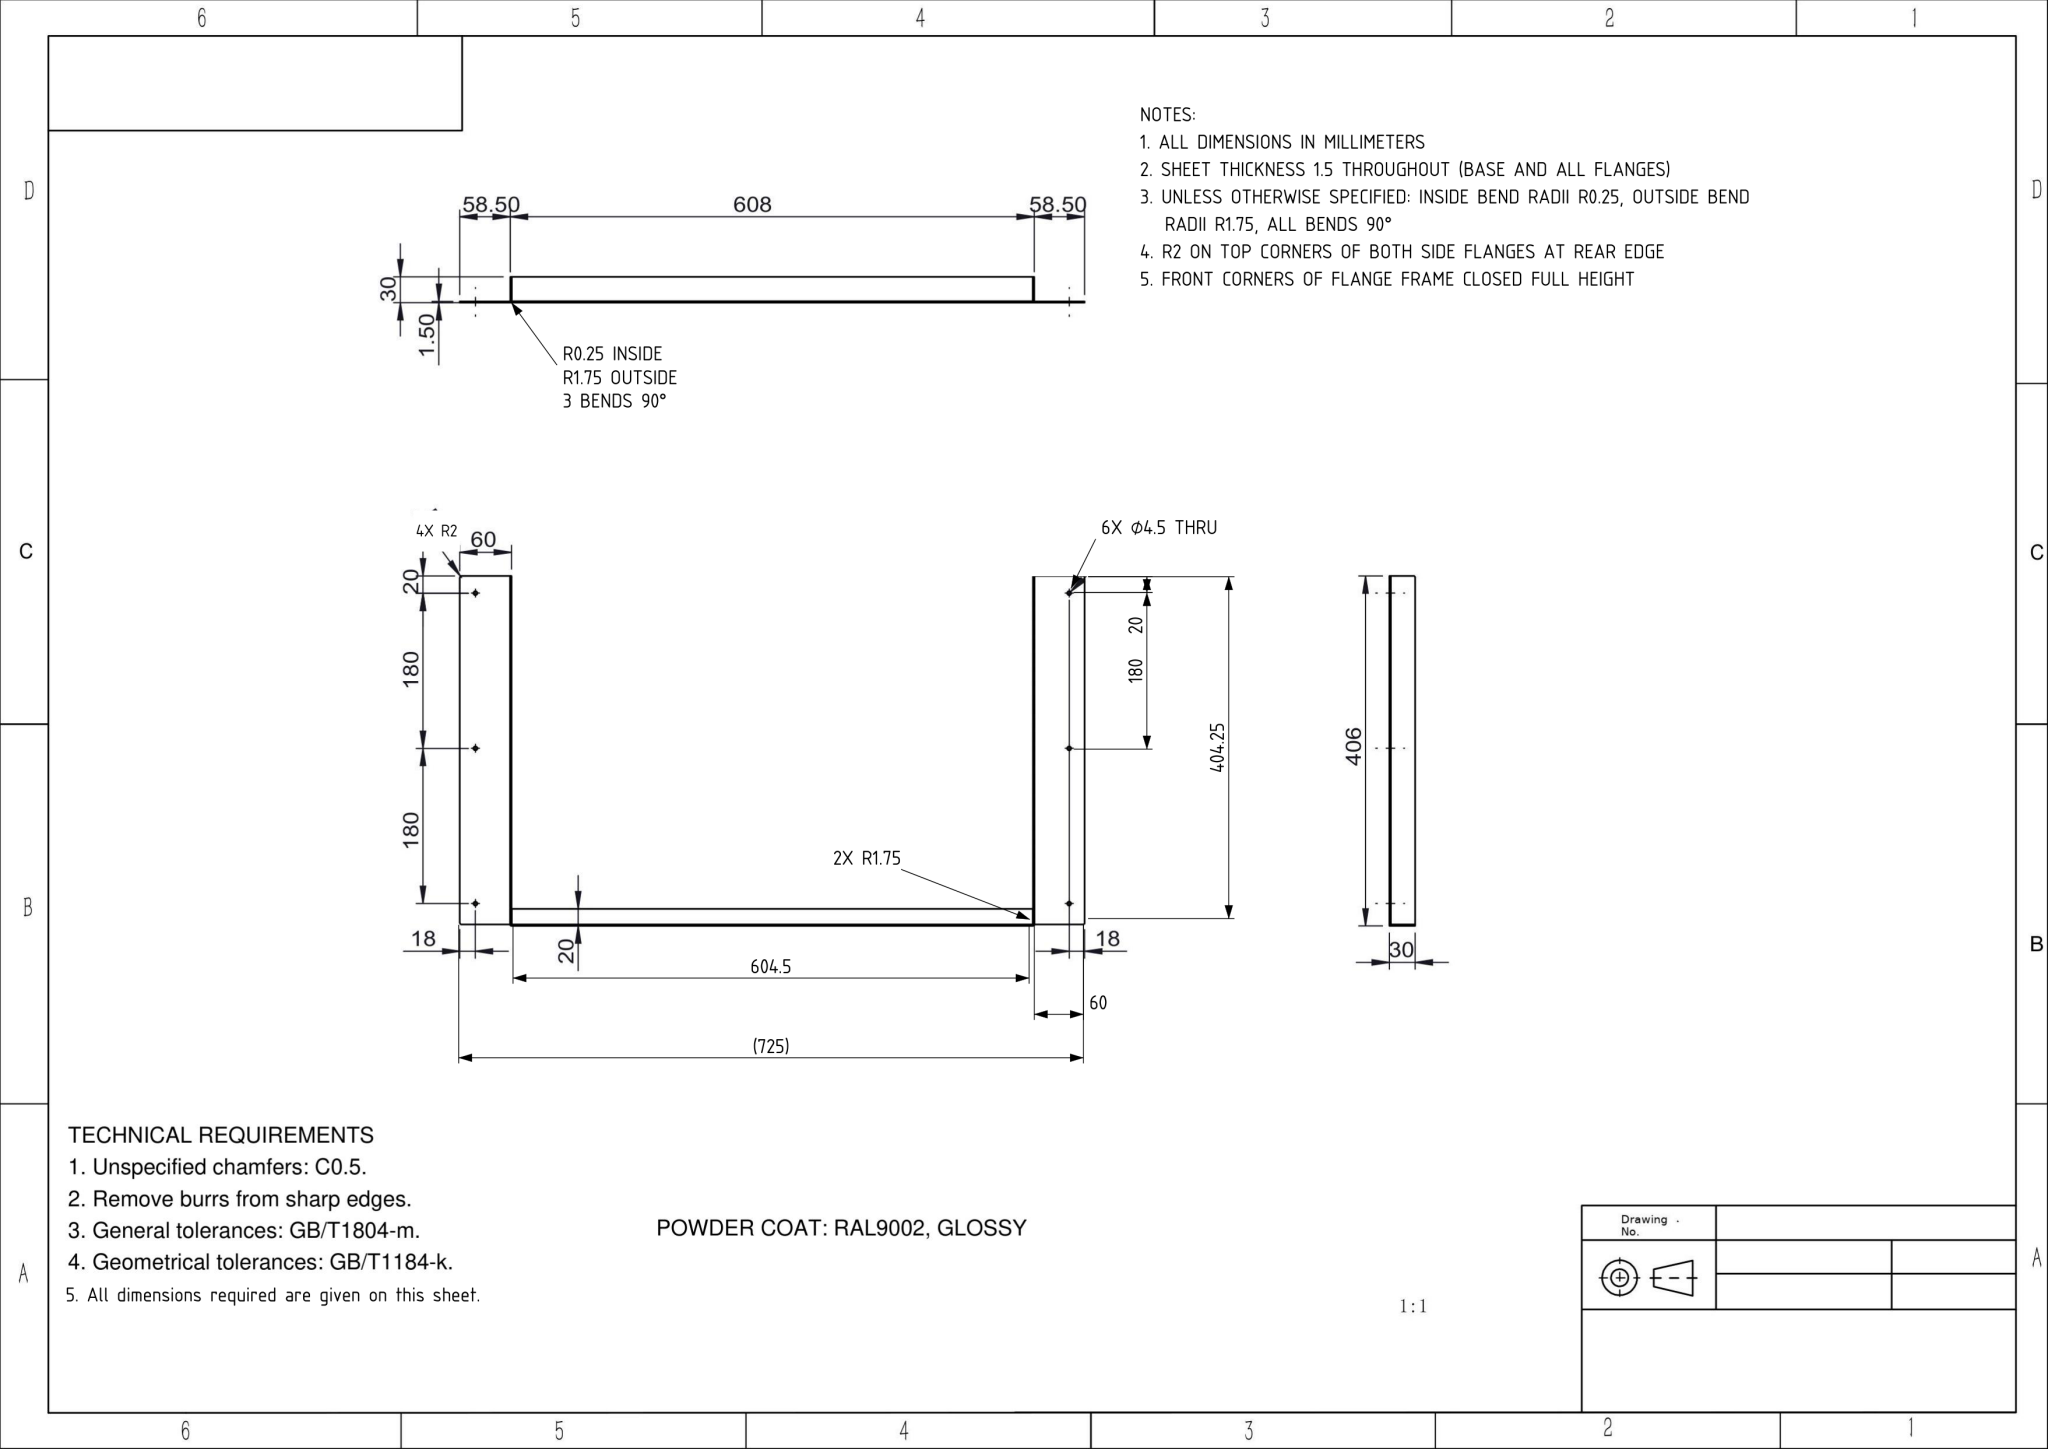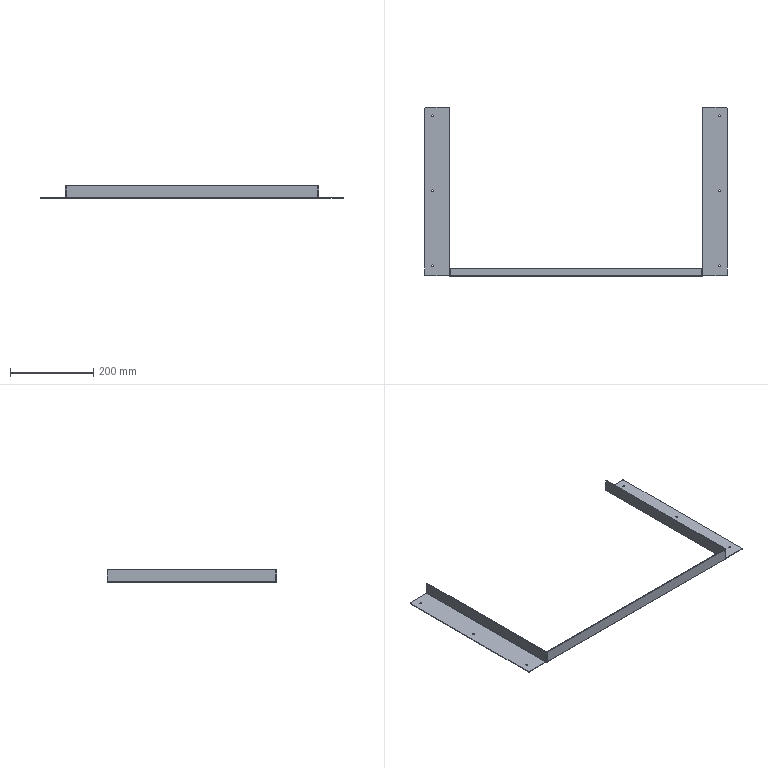Part | NX | mm | 1 solid | 68 faces | box 725 x 406 x 30 mm | volume 150387 mm3 | plane 40 | cylinder 28 | commonest cylinder face diameters 4.5 x12 4 x6 0.5 x5 3.5 x5